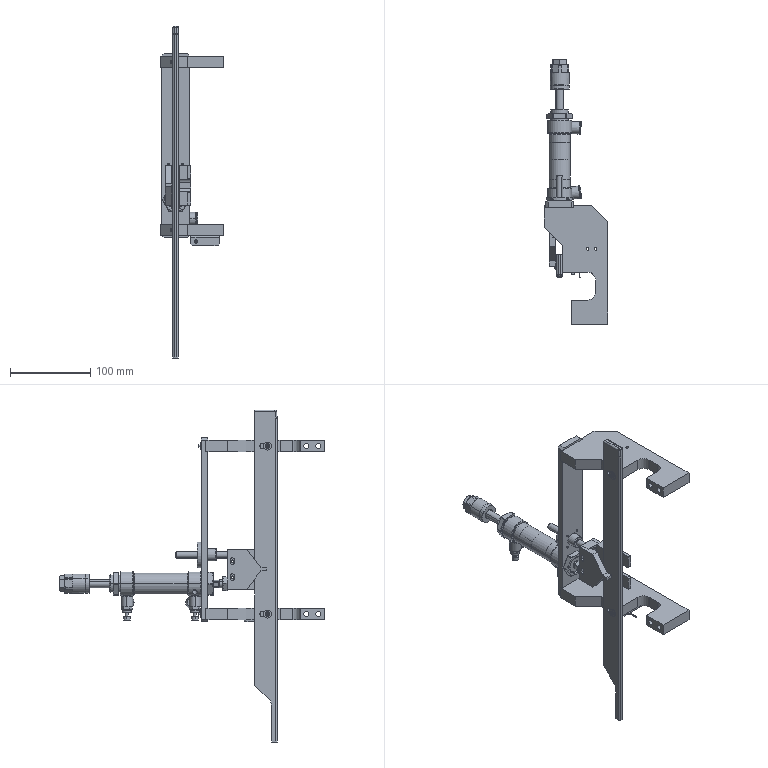Assembly | SolidWorks | mm | 43 component files | 43 solids | 1017 faces | box 79.8 x 330.8 x 415 mm | volume 484823 mm3 | plane 465 | cylinder 355 | cone 152 | torus 36 | spline 5 | sphere 4 | commonest cylinder face diameters 3 x40 10 x30 4.2 x28 5.5 x26 1.6 x22 4 x20 6 x18 8 x14
Bill of materials:
AS2201-01-F06S | 2 |  | Elbow-shaped body made of cylinders: a vertical cylindrical body with a smaller round boss on top and a stepped round stem below, plus a larger cylindrical sleeve coming off the side at right angles, with a central bore and grooves near its open end.
FiberOpticHeadM4x10 | 1 |  | Solid stepped round shaft with four coaxial sections: a long thin end, a short slightly larger step, a large central body, and a medium-diameter section at the other end.
hexagon socket head cap screws gb | 11 |  | Headed cylindrical fastener-like part: a round cylindrical head with rounded edges on a plain round shank with a chamfered tip.
MISUMI Linear Bearing LHFR8 | 1 |  | Flanged bushing: a round flange with four through-holes on a bolt circle, and a cylindrical hub with a central through-bore.
AIRTAC MACJ25x25-10S | 1 |  | Elongated, hollow, stepped cylindrical part (looks like a sleeve or tube). From end to end: a smaller-diameter spigot, a wider collar, a long central cylinder slightly narrower than the collars, a second wider collar, and a second smaller spigot. The steps are roughly symmetric. A round bore runs along the axis, and small local cutouts appear on one side of the collars.
plain washers-n series-grade a gb | 2 |  | Plain flat annular ring (washer shape): a thin disk with a concentric central hole.
plain washers--product grade c gb | 4 |  | Plain flat annular ring (washer shape): a thin disk with a concentric central hole, very similar to the other flat ring.
spring lock washers--normal type gb | 6 |  | Split ring with a rectangular cross-section and one radial cut, offset at an angle (split lock washer shape).
A3 Steel | 1 | A3 Steel | Rectangular block with two larger round through-holes on one face and two smaller round holes on the adjacent face, set at right angles to the larger holes.
Stainless Steel201 | 1 | 201 Stainless Steel | L-shaped bent sheet-metal-style bracket: a long elongated slot in one flange and a single round hole in the other, with chamfered corners.
Cr12 | 1 | 40Cr | Long slender round tube or sleeve with a small central bore and lightly chamfered ends.
Nylon6/10 | 1 | Nylon 6/10 | Rectangular plate with a U-shaped open slot running in from one edge and two round holes near the opposite edge. Its side profile is stepped, with offset tongues projecting from the top and bottom edges.
Nylon6/10 | 1 | Nylon 6/10 | Flat gusset-like plate: a straight back edge with two obround slots, sides tapering to a narrow apex, and a small rectangular tab sticking out from the apex. There is a step in the thickness along the top.
Nylon6/10 | 1 | Nylon 6/10 | Long, thin flat strip of constant thickness. Two oblong slots are spaced along its length. At one end the width steps down along an angled edge into a narrower straight tab.
A3 Steel | 2 | A3 Steel | Solid prismatic block with an irregular stepped outline. One side has a U-shaped notch with rounded inner corners, and the outline also has angled (chamfered) corner edges. There are two small holes in the top face and two larger round bores in one end face.
A3 Steel | 1 | A3 Steel | Flat rectangular plate with chamfered corners. It has two parallel oblong slots at each end, a medium round hole surrounded by four small holes in a square pattern, and a larger round hole near the middle of its length.
Mates:
1. coincident | WirePressingUnitSupportLeg-1 face at (10.665, 64.368, 9.085) dir (0, 1, 0) | WirePressingUnitUpperPlate-1 face at (-4.335, 64.368, -95.515) dir (0, -1, 0)
2. coincident | WirePressingUnitSupportLeg-1 face at (13.065, 64.368, 1.685) dir (-1, 0, 0) | WirePressingUnitUpperPlate-1 face at (13.065, 72.168, 19.485) dir (1, 0, 0)
3. distance | WirePressingUnitUpperPlate-1 face at (-21.735, 72.168, 19.485) dir (0, 0, 1) | WirePressingUnitSupportLeg-1 face at (30.665, -26.632, 16.485) dir (0, 0, 1)
4. coincident | WirePressingUnitUpperPlate-1 face at (-4.335, 72.168, -95.515) dir (0, 1, 0) | LinearBearingLHFR8-1 face at (18.428, 72.168, -126.879) dir (0, -1, 0)
5. concentric | WirePressingUnitUpperPlate-1 face at (-4.335, 64.368, -127.015) dir (0, 1, 0) r 7.5 | LinearBearingLHFR8-1 face at (-4.335, 71.668, -127.015) dir (0, 1, 0) r 7.5
6. concentric | WirePressingUnitUpperPlate-1 face at (4.15, 72.168, -118.53) dir (0, 1, 0) r 1.25 | LinearBearingLHFR8-1 face at (4.15, 72.168, -118.53) dir (0, 1, 0) r 1.75
7. coincident | WirePressingUnitUpperPlate-1 face at (-4.335, 72.168, -95.515) dir (0, 1, 0) | MACJ25x25-10S-Body-1/MACJ25x25-10S-Body-1 face at (-4.335, 72.168, -174.015) dir (0, -1, 0)
8. concentric | WirePressingUnitUpperPlate-1 face at (-4.335, 72.168, -163.015) dir (0, -1, 0) r 11.1 | MACJ25x25-10S-Body-1/MACJ25x25-10S-Body-1 face at (-4.335, 173.168, -163.015) dir (0, -1, 0) r 15
9. parallel | WirePressingUnitSupportLeg-1 face at (30.665, -26.632, 16.485) dir (0, 0, 1) | MACJ25x25-10S-Body-1/25 MA Nut-2 face at (4.036, 64.368, -177.515) dir (0, 0, -1)
10. concentric | LinearBearingLHFR8-1 face at (-4.335, 53.168, -127.015) dir (0, 1, 0) r 4 | WirePressingUnitGuidePost-1 face at (-4.335, 39.168, -127.015) dir (0, 1, 0) r 4
11. coincident | WirePressingUnitCylinderConnectionBlock-1 face at (-4.335, 39.168, -145.015) dir (0, 1, 0) | WirePressingUnitGuidePost-1 face at (-4.335, 39.168, -127.015) dir (0, -1, 0)
12. concentric | MACJ25x25-10S-Rod-1/MACJ25x25-10S-Rod-1 face at (-4.335, 249.168, -163.015) dir (0, -1, 0) r 5 | WirePressingUnitCylinderConnectionBlock-1 face at (-4.335, 27.368, -163.015) dir (0, -1, 0) r 5
13. coincident | MACJ25x25-10S-Rod-1/25 MA Nut1-1 face at (0.1975, 39.168, -155.824) dir (0, -1, 0) | WirePressingUnitCylinderConnectionBlock-1 face at (-4.335, 39.168, -145.015) dir (0, 1, 0)
14. concentric | WirePressingUnitGuidePost-1 face at (-4.335, 39.168, -127.015) dir (0, 1, 0) r 4 | WirePressingUnitCylinderConnectionBlock-1 face at (-4.335, 27.368, -127.015) dir (0, -1, 0) r 5
15. coincident | WirePressingUnitSupportLeg-1 face at (-0.8352, 66.368, 16.485) dir (-1, 0, 0) | WirePressingUnitPressingPlate-1 face at (-0.8352, -8.632, -153.415) dir (1, 0, 0)
16. coincident | WirePressingUnitCylinderConnectionBlock-1 face at (-13.235, 27.368, -120.115) dir (-1, 0, 0) | WirePressingUnitPressingHead-2 face at (-13.235, 27.368, -120.115) dir (1, 0, 0)
17. concentric | WirePressingUnitCylinderConnectionBlock-1 face at (-13.235, 33.268, -155.015) dir (-1, 0, 0) r 1.65 | WirePressingUnitPressingHead-2 sketch point at (-17.235, 33.268, -155.015) dir (1, 0, 0)
18. concentric | MACJ25x25-10S-Body-1/MACJ25x25-10S-Body-1 face at (-4.335, 165.168, -170.015) dir (0, 0, -1) r 4.865 | AS2201-01-F06S-1 face at (-4.335, 165.168, -172.595) dir (0, 0, 1) r 4.865
19. distance | AS2201-01-F06S-1 face at (-8.838, 161.059, -172.015) dir (0, 0, 1) | MACJ25x25-10S-Body-1/MACJ25x25-10S-Body-1 face at (-4.335, 170.033, -170.015) dir (0, 0, -1)
20. coincident | AS2201-01-F06S-1 face at (-0.5494, 160.919, -208.415) dir (0, 0, -1) | AS2201-01-F06S-2 face at (0.1957, 76.725, -208.415) dir (0, 0, -1)
21. concentric | MACJ25x25-10S-Body-1/MACJ25x25-10S-Body-1 face at (-4.335, 80.168, -170.015) dir (0, 0, -1) r 4.865 | AS2201-01-F06S-2 face at (-4.335, 80.168, -172.595) dir (0, 0, 1) r 4.865
22. coincident | WirePressingUnitSupportLeg-3 face at (30.665, -26.632, -208.315) dir (0, 0, -1) | WirePressingUnitFiberOpticBracket-1 face at (14.665, -4.632, -208.315) dir (0, 0, 1)
23. concentric | WirePressingUnitSupportLeg-3 face at (40.665, 12.368, -208.315) dir (0, 0, -1) r 1.65 | WirePressingUnitFiberOpticBracket-1 sketch point at (40.665, 12.368, -210.315) dir (1, 0, 0)
24. concentric | WirePressingUnitSupportLeg-3 face at (30.665, 12.368, -208.315) dir (0, 0, -1) r 1.65 | WirePressingUnitFiberOpticBracket-1 sketch point at (30.665, 12.368, -210.315) dir (1, 0, 0)
25. concentric | WirePressingUnitFiberOpticBracket-1 face at (20.665, -6.632, -215.315) dir (0, -1, 0) r 2 | FiberOpticHeadM4x10-1 face at (20.665, -23.632, -215.315) dir (0, 1, 0) r 2
26. distance | FiberOpticHeadM4x10-1 face at (20.665, -23.632, -215.315) dir (0, -1, 0) | WirePressingUnitFiberOpticBracket-1 face at (14.665, -6.632, -220.315) dir (0, -1, 0)
27. concentric | WirePressingUnitCylinderConnectionBlock-1 face at (-4.335, 27.368, -127.015) dir (0, -1, 0) r 2.75 | hexagon socket head cap screws gb-5 face at (-4.335, 38.868, -127.015) dir (0, -1, 0) r 0.8
28. coincident | WirePressingUnitCylinderConnectionBlock-1 face at (-4.335, 32.868, -129.765) dir (0, -1, 0) | hexagon socket head cap screws gb-5 face at (-4.335, 32.868, -127.015) dir (0, 1, 0)
29. coincident | WirePressingUnitPressingPlate-1 face at (-7.835, -8.632, -153.415) dir (-1, 0, 0) | plain washers-n series-grade a gb-1 face at (-7.835, -10.632, 9.085) dir (1, 0, 0)
30. concentric | WirePressingUnitSupportLeg-1 face at (-0.8352, -10.632, 9.085) dir (-1, 0, 0) r 2.5 | plain washers-n series-grade a gb-1 face at (-7.835, -10.632, 9.085) dir (-1, 0, 0) r 2.75
31. coincident | WirePressingUnitPressingPlate-1 face at (-7.835, -8.632, -153.415) dir (-1, 0, 0) | plain washers-n series-grade a gb-3 face at (-7.835, -10.632, -200.915) dir (1, 0, 0)
32. concentric | WirePressingUnitSupportLeg-3 face at (-0.8352, -10.632, -200.915) dir (-1, 0, 0) r 2.5 | plain washers-n series-grade a gb-3 face at (-7.835, -10.632, -200.915) dir (-1, 0, 0) r 2.75
33. concentric | plain washers-n series-grade a gb-3 face at (-7.835, -10.632, -200.915) dir (-1, 0, 0) r 2.75 | spring lock washers--normal type gb-1 face at (-8.835, -10.632, -200.915) dir (-1, 0, 0) r 1.5
34. coincident | plain washers-n series-grade a gb-3 face at (-8.835, -10.632, -200.915) dir (-1, 0, 0) | spring lock washers--normal type gb-1 face at (-8.835, -10.632, -200.915) dir (1, 0, 0)
35. concentric | plain washers-n series-grade a gb-1 face at (-7.835, -10.632, 9.085) dir (-1, 0, 0) r 2.75 | spring lock washers--normal type gb-2 face at (-8.835, -10.632, 9.085) dir (-1, 0, 0) r 1.5
36. coincident | plain washers-n series-grade a gb-1 face at (-8.835, -10.632, 9.085) dir (-1, 0, 0) | spring lock washers--normal type gb-2 face at (-8.835, -10.632, 9.085) dir (1, 0, 0)
37. concentric | spring lock washers--normal type gb-2 face at (-8.835, -10.632, 9.085) dir (-1, 0, 0) r 2.1 | hexagon socket head cap screws gb-6 face at (-3.435, -10.632, 9.085) dir (-1, 0, 0) r 0.8
38. coincident | spring lock washers--normal type gb-2 face at (-9.435, -10.632, 9.085) dir (-1, 0, 0) | hexagon socket head cap screws gb-6 face at (-9.435, -10.632, 9.085) dir (1, 0, 0)
39. concentric | spring lock washers--normal type gb-1 face at (-8.835, -10.632, -200.915) dir (-1, 0, 0) r 1.5 | hexagon socket head cap screws gb-7 face at (-3.435, -10.632, -200.915) dir (-1, 0, 0) r 0.8
40. coincident | spring lock washers--normal type gb-1 face at (-9.435, -10.632, -200.915) dir (-1, 0, 0) | hexagon socket head cap screws gb-7 face at (-9.435, -10.632, -200.915) dir (1, 0, 0)
41. concentric | LinearBearingLHFR8-1 face at (-12.82, 74.068, -118.53) dir (0, 1, 0) r 3 | hexagon socket head cap screws gb-8 face at (-12.82, 68.068, -118.53) dir (0, 1, 0) r 0.8
42. coincident | LinearBearingLHFR8-1 face at (-12.795, 74.068, -114.261) dir (0, 1, 0) | hexagon socket head cap screws gb-8 face at (-12.82, 74.068, -118.53) dir (0, -1, 0)
43. concentric | LinearBearingLHFR8-1 face at (4.15, 74.068, -118.53) dir (0, 1, 0) r 3 | hexagon socket head cap screws gb-9 face at (4.15, 68.068, -118.53) dir (0, 1, 0) r 0.8
44. coincident | LinearBearingLHFR8-1 face at (4.176, 74.068, -114.261) dir (0, 1, 0) | hexagon socket head cap screws gb-9 face at (4.15, 74.068, -118.53) dir (0, -1, 0)
45. concentric | LinearBearingLHFR8-1 face at (4.15, 74.068, -135.5) dir (0, 1, 0) r 3 | hexagon socket head cap screws gb-10 face at (4.15, 68.068, -135.5) dir (0, 1, 0) r 0.8
46. coincident | LinearBearingLHFR8-1 face at (4.176, 74.068, -131.232) dir (0, 1, 0) | hexagon socket head cap screws gb-10 face at (4.15, 74.068, -135.5) dir (0, -1, 0)
47. concentric | LinearBearingLHFR8-1 face at (-12.82, 74.068, -135.5) dir (0, 1, 0) r 3 | hexagon socket head cap screws gb-11 face at (-12.82, 68.068, -135.5) dir (0, 1, 0) r 0.8
48. coincident | LinearBearingLHFR8-1 face at (-12.795, 74.068, -131.232) dir (0, 1, 0) | hexagon socket head cap screws gb-11 face at (-12.82, 74.068, -135.5) dir (0, -1, 0)
49. coincident | WirePressingUnitUpperPlate-1 face at (-4.335, 72.168, -95.515) dir (0, 1, 0) | plain washers--product grade c gb-2 face at (-14.335, 72.168, 9.085) dir (0, -1, 0)
50. concentric | WirePressingUnitSupportLeg-1 face at (-14.335, 64.368, 9.085) dir (0, 1, 0) r 2.1 | plain washers--product grade c gb-2 face at (-14.335, 73.168, 9.085) dir (0, -1, 0) r 2.75
51. coincident | WirePressingUnitUpperPlate-1 face at (-4.335, 72.168, -95.515) dir (0, 1, 0) | plain washers--product grade c gb-3 face at (5.665, 72.168, 9.085) dir (0, -1, 0)
52. concentric | WirePressingUnitSupportLeg-1 face at (5.665, 64.368, 9.085) dir (0, 1, 0) r 2.1 | plain washers--product grade c gb-3 face at (5.665, 73.168, 9.085) dir (0, -1, 0) r 2.75
53. coincident | WirePressingUnitUpperPlate-1 face at (-4.335, 72.168, -95.515) dir (0, 1, 0) | plain washers--product grade c gb-4 face at (5.665, 72.168, -200.915) dir (0, -1, 0)
54. concentric | WirePressingUnitSupportLeg-3 face at (5.665, 64.368, -200.915) dir (0, 1, 0) r 2.1 | plain washers--product grade c gb-4 face at (5.665, 73.168, -200.915) dir (0, -1, 0) r 2.75
55. coincident | WirePressingUnitUpperPlate-1 face at (-4.335, 72.168, -95.515) dir (0, 1, 0) | plain washers--product grade c gb-5 face at (-14.335, 72.168, -200.915) dir (0, -1, 0)
56. concentric | WirePressingUnitSupportLeg-3 face at (-14.335, 64.368, -200.915) dir (0, 1, 0) r 2.1 | plain washers--product grade c gb-5 face at (-14.335, 73.168, -200.915) dir (0, -1, 0) r 2.75
57. concentric | plain washers--product grade c gb-2 face at (-14.335, 73.168, 9.085) dir (0, -1, 0) r 2.75 | spring lock washers--normal type gb-3 face at (-14.335, 73.168, 9.085) dir (0, 1, 0) r 1.5
58. coincident | plain washers--product grade c gb-2 face at (-14.335, 73.168, 9.085) dir (0, 1, 0) | spring lock washers--normal type gb-3 face at (-14.335, 73.168, 9.085) dir (0, -1, 0)
59. concentric | plain washers--product grade c gb-3 face at (5.665, 73.168, 9.085) dir (0, -1, 0) r 2.75 | spring lock washers--normal type gb-7 face at (5.665, 73.168, 9.085) dir (0, 1, 0) r 1.5
60. coincident | plain washers--product grade c gb-3 face at (5.665, 73.168, 9.085) dir (0, 1, 0) | spring lock washers--normal type gb-7 face at (5.665, 73.168, 9.085) dir (0, -1, 0)
61. concentric | plain washers--product grade c gb-4 face at (5.665, 73.168, -200.915) dir (0, -1, 0) r 2.75 | spring lock washers--normal type gb-8 face at (5.665, 73.168, -200.915) dir (0, 1, 0) r 1.5
62. coincident | plain washers--product grade c gb-4 face at (5.665, 73.168, -200.915) dir (0, 1, 0) | spring lock washers--normal type gb-8 face at (5.665, 73.168, -200.915) dir (0, -1, 0)
63. concentric | plain washers--product grade c gb-5 face at (-14.335, 73.168, -200.915) dir (0, -1, 0) r 2.75 | spring lock washers--normal type gb-9 face at (-14.335, 73.168, -200.915) dir (0, 1, 0) r 1.5
64. coincident | plain washers--product grade c gb-5 face at (-14.335, 73.168, -200.915) dir (0, 1, 0) | spring lock washers--normal type gb-9 face at (-14.335, 73.168, -200.915) dir (0, -1, 0)
65. concentric | spring lock washers--normal type gb-7 face at (5.665, 73.168, 9.085) dir (0, 1, 0) r 2.1 | hexagon socket head cap screws gb-12 face at (5.665, 67.768, 9.085) dir (0, 1, 0) r 0.8
66. coincident | spring lock washers--normal type gb-7 face at (5.665, 73.768, 9.085) dir (0, 1, 0) | hexagon socket head cap screws gb-12 face at (5.665, 73.768, 9.085) dir (0, -1, 0)
67. concentric | spring lock washers--normal type gb-3 face at (-14.335, 73.168, 9.085) dir (0, 1, 0) r 1.5 | hexagon socket head cap screws gb-2 face at (-14.335, 67.768, 9.085) dir (0, 1, 0) r 0.8
68. coincident | spring lock washers--normal type gb-3 face at (-14.335, 73.768, 9.085) dir (0, 1, 0) | hexagon socket head cap screws gb-2 face at (-14.335, 73.768, 9.085) dir (0, -1, 0)
69. concentric | spring lock washers--normal type gb-8 face at (5.665, 73.168, -200.915) dir (0, 1, 0) r 1.5 | hexagon socket head cap screws gb-3 face at (5.665, 67.768, -200.915) dir (0, 1, 0) r 0.8
70. coincident | spring lock washers--normal type gb-8 face at (5.665, 73.768, -200.915) dir (0, 1, 0) | hexagon socket head cap screws gb-3 face at (5.665, 73.768, -200.915) dir (0, -1, 0)
71. concentric | spring lock washers--normal type gb-9 face at (-14.335, 73.168, -200.915) dir (0, 1, 0) r 1.5 | hexagon socket head cap screws gb-4 face at (-14.335, 67.768, -200.915) dir (0, 1, 0) r 0.8
72. coincident | spring lock washers--normal type gb-9 face at (-14.335, 73.768, -200.915) dir (0, 1, 0) | hexagon socket head cap screws gb-4 face at (-14.335, 73.768, -200.915) dir (0, -1, 0)
73. concentric | WirePressingUnitSupportLeg-1 face at (-0.8352, -10.632, 9.085) dir (-1, 0, 0) r 2.5 | WirePressingUnitPressingPlate-1 face at (2.165, -10.632, 9.085) dir (-1, 0, 0) r 3.5
74. concentric | WirePressingUnitPressingPlate-1 face at (2.165, -10.632, -200.915) dir (-1, 0, 0) r 3.5 | hexagon socket head cap screws gb-7 face at (-3.435, -10.632, -200.915) dir (-1, 0, 0) r 0.8
75. coincident | WirePressingUnitCylinderConnectionBlock-1 face at (4.565, 27.368, -120.115) dir (1, 0, 0) | WirePressingUnitLocatingPlate-1 face at (4.565, 27.368, -169.915) dir (-1, 0, 0)
76. concentric | WirePressingUnitCylinderConnectionBlock-1 face at (-13.235, 33.268, -155.015) dir (-1, 0, 0) r 1.65 | WirePressingUnitLocatingPlate-1 face at (4.565, 33.268, -155.015) dir (1, 0, 0) r 2.25
77. concentric | WirePressingUnitCylinderConnectionBlock-1 face at (-13.235, 33.268, -135.015) dir (-1, 0, 0) r 1.65 | WirePressingUnitLocatingPlate-1 face at (4.565, 33.268, -135.015) dir (1, 0, 0) r 2.25
78. distance | MACJ25x25-10S-Rod-1/MACJ25x25-10S-Rod-1 face at (-10.868, 146.168, -173.378) dir (0, 1, 0) | MACJ25x25-10S-Body-1/MACJ25x25-10S-Body-1 face at (-4.335, 146.168, -175.515) dir (0, -1, 0)
79. concentric | MACJ25x25-10S-Body-1/MACJ25x25-10S-Body-1 face at (-4.335, 187.168, -163.015) dir (0, -1, 0) r 12.5 | MACJ25x25-10S-Rod-1/MACJ25x25-10S-Rod-1 face at (-4.335, 249.168, -163.015) dir (0, -1, 0) r 12.25
80. concentric | WirePressingUnitCylinderConnectionBlock-1 face at (-13.235, 33.268, -135.015) dir (-1, 0, 0) r 1.65 | WirePressingUnitPressingHead-2 sketch point at (-17.235, 33.268, -135.015) dir (1, 0, 0)
81. distance | MACJ25x25-10S-Body-1 face at (-16, 0, 11) dir (-1, 0, 0) | 25 MA Nut-2 face at (-23.8, 14.2, 0) dir (1, 0, 0)
82. concentric | MACJ25x25-10S-Body-1 face at (85, 0, 0) dir (-1, 0, 0) r 11 | 25 MA Nut-2 face at (-23.8, 0, 0) dir (-1, 0, 0) r 11
83. distance | MACJ25x25-10S-Body-1 face at (85, 0, 14.6) dir (1, 0, 0) | 25 MA Nut-1 face at (87, 14.2, 0) dir (-1, 0, 0)
84. concentric | MACJ25x25-10S-Body-1 face at (99, 0, 0) dir (-1, 0, 0) r 11 | 25 MA Nut-1 face at (87, 0, 0) dir (1, 0, 0) r 11
85. concentric | MACJ25x25-10S-Rod-1 face at (161, 0, 0) dir (-1, 0, 0) r 5 | 25 MAJ Nut-1 face at (161, 0, 0) dir (-1, 0, 0) r 5
86. coincident | MACJ25x25-10S-Rod-1 face at (161, 4.233, 0) dir (1, 0, 0) | 25 MAJ Nut-1 face at (161, 0, 8.5) dir (1, 0, 0)
87. concentric | MACJ25x25-10S-Rod-1 face at (161, 0, 0) dir (-1, 0, 0) r 5 | 25MACJ2510A-Nut-1 face at (155, 0, 0) dir (-1, 0, 0) r 5
88. coincident | 25 MAJ Nut-1 face at (155, 0, 0) dir (-1, 0, 0) | 25MACJ2510A-Nut-1 face at (155, 0, 10.5) dir (1, 0, 0)
89. concentric | MACJ25x25-10S-Rod-1 face at (161, 0, 0) dir (-1, 0, 0) r 5 | 25 MA Nut1-1 face at (-49, 0, 0) dir (1, 0, 0) r 5
90. distance | 25 MA Nut1-1 face at (-49, -8.5, 0) dir (-1, 0, 0) | MACJ25x25-10S-Rod-1 face at (-60, 0, 0) dir (-1, 0, 0)